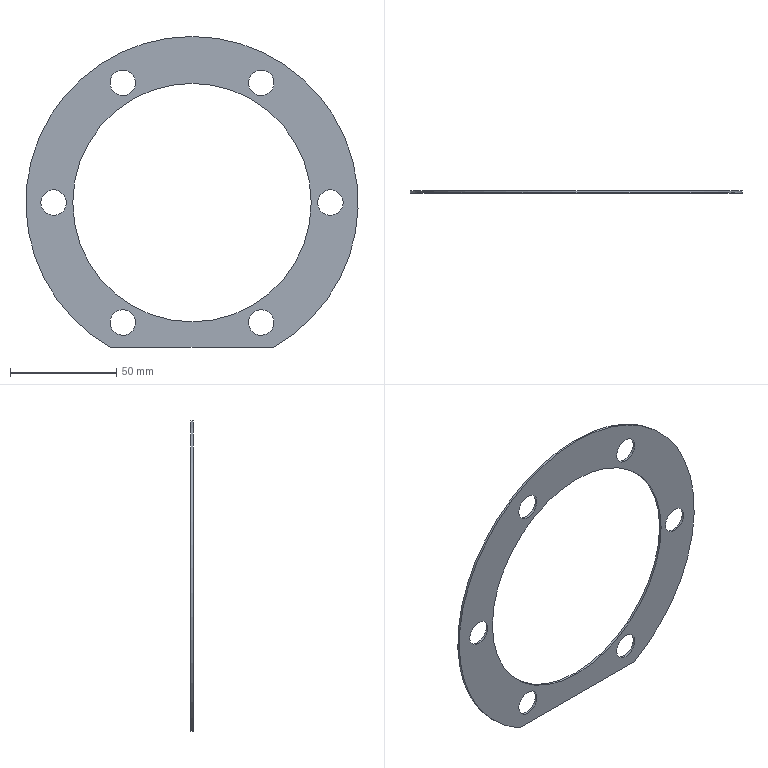Component | NX | T1_GASKET | 1 solid | 11 faces | box 156 x 1 x 146 mm | volume 8066 mm3 | cylinder 8 | plane 3 | commonest cylinder face diameters 12 x6 112 x1 156 x1
STEP:
#1=CARTESIAN_POINT('',(0.,0.,0.));
#2=DIRECTION('',(0.,0.,1.));
#3=DIRECTION('',(1.,0.,0.));
#4=AXIS2_PLACEMENT_3D('',#1,#2,#3);
#5=CARTESIAN_POINT('',(-41.21,121.,-71.));
#6=VERTEX_POINT('',#5);
#7=CARTESIAN_POINT('',(35.21,121.,-71.));
#8=VERTEX_POINT('',#7);
#9=CARTESIAN_POINT('',(-41.21,121.,-71.));
#10=DIRECTION('',(1.,0.,0.));
#11=VECTOR('',#10,1.);
#12=LINE('',#9,#11);
#13=CARTESIAN_POINT('',(-41.21,120.,-71.));
#14=DIRECTION('',(0.,0.,1.));
#15=DIRECTION('',(1.,0.,0.));
#16=AXIS2_PLACEMENT_3D('',#13,#14,#15);
#17=PLANE('',#16);
#18=CARTESIAN_POINT('',(0.,1.));
#19=DIRECTION('',(1.,0.));
#20=VECTOR('',#19,1.);
#21=LINE('',#18,#20);
#22=(GEOMETRIC_REPRESENTATION_CONTEXT(2)PARAMETRIC_REPRESENTATION_CONTEXT()REPRESENTATION_CONTEXT('',''));
#23=DEFINITIONAL_REPRESENTATION('',(#21),#22);
#24=PCURVE('',#17,#23);
#25=CARTESIAN_POINT('',(-3.,121.,-3.));
#26=DIRECTION('',(0.,-1.,0.));
#27=DIRECTION('',(0.,0.,-1.));
#28=AXIS2_PLACEMENT_3D('',#25,#26,#27);
#29=PLANE('',#28);
#30=CARTESIAN_POINT('',(68.,-38.21));
#31=DIRECTION('',(0.,1.));
#32=VECTOR('',#31,1.);
#33=LINE('',#30,#32);
#34=(GEOMETRIC_REPRESENTATION_CONTEXT(2)PARAMETRIC_REPRESENTATION_CONTEXT()REPRESENTATION_CONTEXT('',''));
#35=DEFINITIONAL_REPRESENTATION('',(#33),#34);
#36=PCURVE('',#29,#35);
#37=SURFACE_CURVE('',#12,(#24,#36),.PCURVE_S1.);
#38=EDGE_CURVE('',#6,#8,#37,.T.);
#39=ORIENTED_EDGE('',*,*,#38,.T.);
#40=CARTESIAN_POINT('',(35.21,120.,-71.));
#41=VERTEX_POINT('',#40);
#42=CARTESIAN_POINT('',(35.21,120.,-71.));
#43=DIRECTION('',(0.,1.,0.));
#44=VECTOR('',#43,1.);
#45=LINE('',#42,#44);
#46=CARTESIAN_POINT('',(76.42,0.));
#47=DIRECTION('',(0.,1.));
#48=VECTOR('',#47,1.);
#49=LINE('',#46,#48);
#50=(GEOMETRIC_REPRESENTATION_CONTEXT(2)PARAMETRIC_REPRESENTATION_CONTEXT()REPRESENTATION_CONTEXT('',''));
#51=DEFINITIONAL_REPRESENTATION('',(#49),#50);
#52=PCURVE('',#17,#51);
#53=CARTESIAN_POINT('',(-3.,120.,-3.));
#54=DIRECTION('',(0.,1.,0.));
#55=DIRECTION('',(0.,0.,1.));
#56=AXIS2_PLACEMENT_3D('',#53,#54,#55);
#57=CYLINDRICAL_SURFACE('',#56,78.);
#58=CARTESIAN_POINT('',(2.63,0.));
#59=DIRECTION('',(0.,1.));
#60=VECTOR('',#59,1.);
#61=LINE('',#58,#60);
#62=(GEOMETRIC_REPRESENTATION_CONTEXT(2)PARAMETRIC_REPRESENTATION_CONTEXT()REPRESENTATION_CONTEXT('',''));
#63=DEFINITIONAL_REPRESENTATION('',(#61),#62);
#64=PCURVE('',#57,#63);
#65=SURFACE_CURVE('',#45,(#52,#64),.PCURVE_S1.);
#66=EDGE_CURVE('',#41,#8,#65,.T.);
#67=ORIENTED_EDGE('',*,*,#66,.F.);
#68=CARTESIAN_POINT('',(-41.21,120.,-71.));
#69=VERTEX_POINT('',#68);
#70=CARTESIAN_POINT('',(-41.21,120.,-71.));
#71=DIRECTION('',(1.,0.,0.));
#72=VECTOR('',#71,1.);
#73=LINE('',#70,#72);
#74=CARTESIAN_POINT('',(0.,0.));
#75=DIRECTION('',(1.,0.));
#76=VECTOR('',#75,1.);
#77=LINE('',#74,#76);
#78=(GEOMETRIC_REPRESENTATION_CONTEXT(2)PARAMETRIC_REPRESENTATION_CONTEXT()REPRESENTATION_CONTEXT('',''));
#79=DEFINITIONAL_REPRESENTATION('',(#77),#78);
#80=PCURVE('',#17,#79);
#81=CARTESIAN_POINT('',(-3.,120.,-3.));
#82=DIRECTION('',(0.,-1.,0.));
#83=DIRECTION('',(0.,0.,-1.));
#84=AXIS2_PLACEMENT_3D('',#81,#82,#83);
#85=PLANE('',#84);
#86=CARTESIAN_POINT('',(68.,-38.21));
#87=DIRECTION('',(0.,1.));
#88=VECTOR('',#87,1.);
#89=LINE('',#86,#88);
#90=(GEOMETRIC_REPRESENTATION_CONTEXT(2)PARAMETRIC_REPRESENTATION_CONTEXT()REPRESENTATION_CONTEXT('',''));
#91=DEFINITIONAL_REPRESENTATION('',(#89),#90);
#92=PCURVE('',#85,#91);
#93=SURFACE_CURVE('',#73,(#80,#92),.PCURVE_S1.);
#94=EDGE_CURVE('',#69,#41,#93,.T.);
#95=ORIENTED_EDGE('',*,*,#94,.F.);
#96=CARTESIAN_POINT('',(-41.21,120.,-71.));
#97=DIRECTION('',(0.,-1.,0.));
#98=VECTOR('',#97,1.);
#99=LINE('',#96,#98);
#100=CARTESIAN_POINT('',(0.,0.));
#101=DIRECTION('',(0.,-1.));
#102=VECTOR('',#101,1.);
#103=LINE('',#100,#102);
#104=(GEOMETRIC_REPRESENTATION_CONTEXT(2)PARAMETRIC_REPRESENTATION_CONTEXT()REPRESENTATION_CONTEXT('',''));
#105=DEFINITIONAL_REPRESENTATION('',(#103),#104);
#106=PCURVE('',#17,#105);
#107=CARTESIAN_POINT('',(-2.63,0.));
#108=DIRECTION('',(0.,-1.));
#109=VECTOR('',#108,1.);
#110=LINE('',#107,#109);
#111=(GEOMETRIC_REPRESENTATION_CONTEXT(2)PARAMETRIC_REPRESENTATION_CONTEXT()REPRESENTATION_CONTEXT('',''));
#112=DEFINITIONAL_REPRESENTATION('',(#110),#111);
#113=PCURVE('',#57,#112);
#114=SURFACE_CURVE('',#99,(#106,#113),.PCURVE_S1.);
#115=EDGE_CURVE('',#6,#69,#114,.T.);
#116=ORIENTED_EDGE('',*,*,#115,.F.);
#117=EDGE_LOOP('',(#39,#67,#95,#116));
#118=FACE_BOUND('',#117,.T.);
#119=ADVANCED_FACE('',(#118),#17,.F.);
#120=CARTESIAN_POINT('',(32.5,120.,-64.488));
#121=VERTEX_POINT('',#120);
#122=CARTESIAN_POINT('',(29.5,120.,-59.292));
#123=DIRECTION('',(0.,-1.,0.));
#124=DIRECTION('',(0.5,0.,-0.866));
#125=AXIS2_PLACEMENT_3D('',#122,#123,#124);
#126=CIRCLE('',#125,6.);
#127=CARTESIAN_POINT('',(29.5,120.,-59.292));
#128=DIRECTION('',(0.,1.,0.));
#129=DIRECTION('',(0.,0.,1.));
#130=AXIS2_PLACEMENT_3D('',#127,#128,#129);
#131=CYLINDRICAL_SURFACE('',#130,6.);
#132=CARTESIAN_POINT('',(8.901,0.));
#133=DIRECTION('',(-1.,0.));
#134=VECTOR('',#133,1.);
#135=LINE('',#132,#134);
#136=(GEOMETRIC_REPRESENTATION_CONTEXT(2)PARAMETRIC_REPRESENTATION_CONTEXT()REPRESENTATION_CONTEXT('',''));
#137=DEFINITIONAL_REPRESENTATION('',(#135),#136);
#138=PCURVE('',#131,#137);
#139=CARTESIAN_POINT('',(56.292,32.5));
#140=DIRECTION('',(0.866,0.5));
#141=AXIS2_PLACEMENT_2D('',#139,#140);
#142=CIRCLE('',#141,6.);
#143=(GEOMETRIC_REPRESENTATION_CONTEXT(2)PARAMETRIC_REPRESENTATION_CONTEXT()REPRESENTATION_CONTEXT('',''));
#144=DEFINITIONAL_REPRESENTATION('',(#142),#143);
#145=PCURVE('',#85,#144);
#146=SURFACE_CURVE('',#126,(#138,#145),.PCURVE_S1.);
#147=EDGE_CURVE('',#121,#121,#146,.T.);
#148=ORIENTED_EDGE('',*,*,#147,.F.);
#149=CARTESIAN_POINT('',(32.5,121.,-64.488));
#150=VERTEX_POINT('',#149);
#151=CARTESIAN_POINT('',(32.5,120.,-64.488));
#152=CARTESIAN_POINT('',(32.5,121.,-64.488));
#153=B_SPLINE_CURVE_WITH_KNOTS('',1,(#151,#152),.UNSPECIFIED.,.F.,.F.,(2,2),(0.,1.),.PIECEWISE_BEZIER_KNOTS.);
#154=CARTESIAN_POINT('',(8.901,0.));
#155=DIRECTION('',(0.,1.));
#156=VECTOR('',#155,1.);
#157=LINE('',#154,#156);
#158=(GEOMETRIC_REPRESENTATION_CONTEXT(2)PARAMETRIC_REPRESENTATION_CONTEXT()REPRESENTATION_CONTEXT('',''));
#159=DEFINITIONAL_REPRESENTATION('',(#157),#158);
#160=PCURVE('',#131,#159);
#161=CARTESIAN_POINT('',(2.618,0.));
#162=DIRECTION('',(0.,1.));
#163=VECTOR('',#162,1.);
#164=LINE('',#161,#163);
#165=(GEOMETRIC_REPRESENTATION_CONTEXT(2)PARAMETRIC_REPRESENTATION_CONTEXT()REPRESENTATION_CONTEXT('',''));
#166=DEFINITIONAL_REPRESENTATION('',(#164),#165);
#167=PCURVE('',#131,#166);
#168=SEAM_CURVE('',#153,(#160,#167),.PCURVE_S1.);
#169=EDGE_CURVE('',#121,#150,#168,.T.);
#170=ORIENTED_EDGE('',*,*,#169,.T.);
#171=CARTESIAN_POINT('',(29.5,121.,-59.292));
#172=DIRECTION('',(0.,-1.,0.));
#173=DIRECTION('',(0.5,0.,-0.866));
#174=AXIS2_PLACEMENT_3D('',#171,#172,#173);
#175=CIRCLE('',#174,6.);
#176=CARTESIAN_POINT('',(8.901,1.));
#177=DIRECTION('',(-1.,0.));
#178=VECTOR('',#177,1.);
#179=LINE('',#176,#178);
#180=(GEOMETRIC_REPRESENTATION_CONTEXT(2)PARAMETRIC_REPRESENTATION_CONTEXT()REPRESENTATION_CONTEXT('',''));
#181=DEFINITIONAL_REPRESENTATION('',(#179),#180);
#182=PCURVE('',#131,#181);
#183=CARTESIAN_POINT('',(56.292,32.5));
#184=DIRECTION('',(0.866,0.5));
#185=AXIS2_PLACEMENT_2D('',#183,#184);
#186=CIRCLE('',#185,6.);
#187=(GEOMETRIC_REPRESENTATION_CONTEXT(2)PARAMETRIC_REPRESENTATION_CONTEXT()REPRESENTATION_CONTEXT('',''));
#188=DEFINITIONAL_REPRESENTATION('',(#186),#187);
#189=PCURVE('',#29,#188);
#190=SURFACE_CURVE('',#175,(#182,#189),.PCURVE_S1.);
#191=EDGE_CURVE('',#150,#150,#190,.T.);
#192=ORIENTED_EDGE('',*,*,#191,.T.);
#193=ORIENTED_EDGE('',*,*,#169,.F.);
#194=EDGE_LOOP('',(#148,#170,#192,#193));
#195=FACE_BOUND('',#194,.F.);
#196=ADVANCED_FACE('',(#195),#131,.F.);
#197=CARTESIAN_POINT('',(-38.5,120.,-64.488));
#198=VERTEX_POINT('',#197);
#199=CARTESIAN_POINT('',(-35.5,120.,-59.292));
#200=DIRECTION('',(0.,-1.,0.));
#201=DIRECTION('',(-0.5,0.,-0.866));
#202=AXIS2_PLACEMENT_3D('',#199,#200,#201);
#203=CIRCLE('',#202,6.);
#204=CARTESIAN_POINT('',(-35.5,120.,-59.292));
#205=DIRECTION('',(0.,1.,0.));
#206=DIRECTION('',(0.,0.,1.));
#207=AXIS2_PLACEMENT_3D('',#204,#205,#206);
#208=CYLINDRICAL_SURFACE('',#207,6.);
#209=CARTESIAN_POINT('',(9.948,0.));
#210=DIRECTION('',(-1.,0.));
#211=VECTOR('',#210,1.);
#212=LINE('',#209,#211);
#213=(GEOMETRIC_REPRESENTATION_CONTEXT(2)PARAMETRIC_REPRESENTATION_CONTEXT()REPRESENTATION_CONTEXT('',''));
#214=DEFINITIONAL_REPRESENTATION('',(#212),#213);
#215=PCURVE('',#208,#214);
#216=CARTESIAN_POINT('',(56.292,-32.5));
#217=DIRECTION('',(0.866,-0.5));
#218=AXIS2_PLACEMENT_2D('',#216,#217);
#219=CIRCLE('',#218,6.);
#220=(GEOMETRIC_REPRESENTATION_CONTEXT(2)PARAMETRIC_REPRESENTATION_CONTEXT()REPRESENTATION_CONTEXT('',''));
#221=DEFINITIONAL_REPRESENTATION('',(#219),#220);
#222=PCURVE('',#85,#221);
#223=SURFACE_CURVE('',#203,(#215,#222),.PCURVE_S1.);
#224=EDGE_CURVE('',#198,#198,#223,.T.);
#225=ORIENTED_EDGE('',*,*,#224,.F.);
#226=CARTESIAN_POINT('',(-38.5,121.,-64.488));
#227=VERTEX_POINT('',#226);
#228=CARTESIAN_POINT('',(-38.5,120.,-64.488));
#229=CARTESIAN_POINT('',(-38.5,121.,-64.488));
#230=B_SPLINE_CURVE_WITH_KNOTS('',1,(#228,#229),.UNSPECIFIED.,.F.,.F.,(2,2),(0.,1.),.PIECEWISE_BEZIER_KNOTS.);
#231=CARTESIAN_POINT('',(9.948,0.));
#232=DIRECTION('',(0.,1.));
#233=VECTOR('',#232,1.);
#234=LINE('',#231,#233);
#235=(GEOMETRIC_REPRESENTATION_CONTEXT(2)PARAMETRIC_REPRESENTATION_CONTEXT()REPRESENTATION_CONTEXT('',''));
#236=DEFINITIONAL_REPRESENTATION('',(#234),#235);
#237=PCURVE('',#208,#236);
#238=CARTESIAN_POINT('',(3.665,0.));
#239=DIRECTION('',(0.,1.));
#240=VECTOR('',#239,1.);
#241=LINE('',#238,#240);
#242=(GEOMETRIC_REPRESENTATION_CONTEXT(2)PARAMETRIC_REPRESENTATION_CONTEXT()REPRESENTATION_CONTEXT('',''));
#243=DEFINITIONAL_REPRESENTATION('',(#241),#242);
#244=PCURVE('',#208,#243);
#245=SEAM_CURVE('',#230,(#237,#244),.PCURVE_S1.);
#246=EDGE_CURVE('',#198,#227,#245,.T.);
#247=ORIENTED_EDGE('',*,*,#246,.T.);
#248=CARTESIAN_POINT('',(-35.5,121.,-59.292));
#249=DIRECTION('',(0.,-1.,0.));
#250=DIRECTION('',(-0.5,0.,-0.866));
#251=AXIS2_PLACEMENT_3D('',#248,#249,#250);
#252=CIRCLE('',#251,6.);
#253=CARTESIAN_POINT('',(9.948,1.));
#254=DIRECTION('',(-1.,0.));
#255=VECTOR('',#254,1.);
#256=LINE('',#253,#255);
#257=(GEOMETRIC_REPRESENTATION_CONTEXT(2)PARAMETRIC_REPRESENTATION_CONTEXT()REPRESENTATION_CONTEXT('',''));
#258=DEFINITIONAL_REPRESENTATION('',(#256),#257);
#259=PCURVE('',#208,#258);
#260=CARTESIAN_POINT('',(56.292,-32.5));
#261=DIRECTION('',(0.866,-0.5));
#262=AXIS2_PLACEMENT_2D('',#260,#261);
#263=CIRCLE('',#262,6.);
#264=(GEOMETRIC_REPRESENTATION_CONTEXT(2)PARAMETRIC_REPRESENTATION_CONTEXT()REPRESENTATION_CONTEXT('',''));
#265=DEFINITIONAL_REPRESENTATION('',(#263),#264);
#266=PCURVE('',#29,#265);
#267=SURFACE_CURVE('',#252,(#259,#266),.PCURVE_S1.);
#268=EDGE_CURVE('',#227,#227,#267,.T.);
#269=ORIENTED_EDGE('',*,*,#268,.T.);
#270=ORIENTED_EDGE('',*,*,#246,.F.);
#271=EDGE_LOOP('',(#225,#247,#269,#270));
#272=FACE_BOUND('',#271,.F.);
#273=ADVANCED_FACE('',(#272),#208,.F.);
#274=CARTESIAN_POINT('',(-74.,120.,-3.));
#275=VERTEX_POINT('',#274);
#276=CARTESIAN_POINT('',(-68.,120.,-3.));
#277=DIRECTION('',(0.,-1.,0.));
#278=DIRECTION('',(-1.,0.,0.));
#279=AXIS2_PLACEMENT_3D('',#276,#277,#278);
#280=CIRCLE('',#279,6.);
#281=CARTESIAN_POINT('',(-68.,120.,-3.));
#282=DIRECTION('',(0.,1.,0.));
#283=DIRECTION('',(0.,0.,1.));
#284=AXIS2_PLACEMENT_3D('',#281,#282,#283);
#285=CYLINDRICAL_SURFACE('',#284,6.);
#286=CARTESIAN_POINT('',(10.996,0.));
#287=DIRECTION('',(-1.,0.));
#288=VECTOR('',#287,1.);
#289=LINE('',#286,#288);
#290=(GEOMETRIC_REPRESENTATION_CONTEXT(2)PARAMETRIC_REPRESENTATION_CONTEXT()REPRESENTATION_CONTEXT('',''));
#291=DEFINITIONAL_REPRESENTATION('',(#289),#290);
#292=PCURVE('',#285,#291);
#293=CARTESIAN_POINT('',(0.,-65.));
#294=DIRECTION('',(-0.,-1.));
#295=AXIS2_PLACEMENT_2D('',#293,#294);
#296=CIRCLE('',#295,6.);
#297=(GEOMETRIC_REPRESENTATION_CONTEXT(2)PARAMETRIC_REPRESENTATION_CONTEXT()REPRESENTATION_CONTEXT('',''));
#298=DEFINITIONAL_REPRESENTATION('',(#296),#297);
#299=PCURVE('',#85,#298);
#300=SURFACE_CURVE('',#280,(#292,#299),.PCURVE_S1.);
#301=EDGE_CURVE('',#275,#275,#300,.T.);
#302=ORIENTED_EDGE('',*,*,#301,.F.);
#303=CARTESIAN_POINT('',(-74.,121.,-3.));
#304=VERTEX_POINT('',#303);
#305=CARTESIAN_POINT('',(-74.,120.,-3.));
#306=CARTESIAN_POINT('',(-74.,121.,-3.));
#307=B_SPLINE_CURVE_WITH_KNOTS('',1,(#305,#306),.UNSPECIFIED.,.F.,.F.,(2,2),(0.,1.),.PIECEWISE_BEZIER_KNOTS.);
#308=CARTESIAN_POINT('',(10.996,0.));
#309=DIRECTION('',(0.,1.));
#310=VECTOR('',#309,1.);
#311=LINE('',#308,#310);
#312=(GEOMETRIC_REPRESENTATION_CONTEXT(2)PARAMETRIC_REPRESENTATION_CONTEXT()REPRESENTATION_CONTEXT('',''));
#313=DEFINITIONAL_REPRESENTATION('',(#311),#312);
#314=PCURVE('',#285,#313);
#315=CARTESIAN_POINT('',(4.712,0.));
#316=DIRECTION('',(0.,1.));
#317=VECTOR('',#316,1.);
#318=LINE('',#315,#317);
#319=(GEOMETRIC_REPRESENTATION_CONTEXT(2)PARAMETRIC_REPRESENTATION_CONTEXT()REPRESENTATION_CONTEXT('',''));
#320=DEFINITIONAL_REPRESENTATION('',(#318),#319);
#321=PCURVE('',#285,#320);
#322=SEAM_CURVE('',#307,(#314,#321),.PCURVE_S1.);
#323=EDGE_CURVE('',#275,#304,#322,.T.);
#324=ORIENTED_EDGE('',*,*,#323,.T.);
#325=CARTESIAN_POINT('',(-68.,121.,-3.));
#326=DIRECTION('',(0.,-1.,0.));
#327=DIRECTION('',(-1.,0.,0.));
#328=AXIS2_PLACEMENT_3D('',#325,#326,#327);
#329=CIRCLE('',#328,6.);
#330=CARTESIAN_POINT('',(10.996,1.));
#331=DIRECTION('',(-1.,0.));
#332=VECTOR('',#331,1.);
#333=LINE('',#330,#332);
#334=(GEOMETRIC_REPRESENTATION_CONTEXT(2)PARAMETRIC_REPRESENTATION_CONTEXT()REPRESENTATION_CONTEXT('',''));
#335=DEFINITIONAL_REPRESENTATION('',(#333),#334);
#336=PCURVE('',#285,#335);
#337=CARTESIAN_POINT('',(0.,-65.));
#338=DIRECTION('',(-0.,-1.));
#339=AXIS2_PLACEMENT_2D('',#337,#338);
#340=CIRCLE('',#339,6.);
#341=(GEOMETRIC_REPRESENTATION_CONTEXT(2)PARAMETRIC_REPRESENTATION_CONTEXT()REPRESENTATION_CONTEXT('',''));
#342=DEFINITIONAL_REPRESENTATION('',(#340),#341);
#343=PCURVE('',#29,#342);
#344=SURFACE_CURVE('',#329,(#336,#343),.PCURVE_S1.);
#345=EDGE_CURVE('',#304,#304,#344,.T.);
#346=ORIENTED_EDGE('',*,*,#345,.T.);
#347=ORIENTED_EDGE('',*,*,#323,.F.);
#348=EDGE_LOOP('',(#302,#324,#346,#347));
#349=FACE_BOUND('',#348,.F.);
#350=ADVANCED_FACE('',(#349),#285,.F.);
#351=CARTESIAN_POINT('',(53.,120.,-3.));
#352=VERTEX_POINT('',#351);
#353=CARTESIAN_POINT('',(-3.,120.,-3.));
#354=DIRECTION('',(0.,-1.,0.));
#355=DIRECTION('',(1.,0.,-0.));
#356=AXIS2_PLACEMENT_3D('',#353,#354,#355);
#357=CIRCLE('',#356,56.);
#358=CARTESIAN_POINT('',(-3.,120.,-3.));
#359=DIRECTION('',(0.,1.,0.));
#360=DIRECTION('',(0.,0.,1.));
#361=AXIS2_PLACEMENT_3D('',#358,#359,#360);
#362=CYLINDRICAL_SURFACE('',#361,56.);
#363=CARTESIAN_POINT('',(7.854,0.));
#364=DIRECTION('',(-1.,0.));
#365=VECTOR('',#364,1.);
#366=LINE('',#363,#365);
#367=(GEOMETRIC_REPRESENTATION_CONTEXT(2)PARAMETRIC_REPRESENTATION_CONTEXT()REPRESENTATION_CONTEXT('',''));
#368=DEFINITIONAL_REPRESENTATION('',(#366),#367);
#369=PCURVE('',#362,#368);
#370=CARTESIAN_POINT('',(0.,0.));
#371=DIRECTION('',(0.,1.));
#372=AXIS2_PLACEMENT_2D('',#370,#371);
#373=CIRCLE('',#372,56.);
#374=(GEOMETRIC_REPRESENTATION_CONTEXT(2)PARAMETRIC_REPRESENTATION_CONTEXT()REPRESENTATION_CONTEXT('',''));
#375=DEFINITIONAL_REPRESENTATION('',(#373),#374);
#376=PCURVE('',#85,#375);
#377=SURFACE_CURVE('',#357,(#369,#376),.PCURVE_S1.);
#378=EDGE_CURVE('',#352,#352,#377,.T.);
#379=ORIENTED_EDGE('',*,*,#378,.F.);
#380=CARTESIAN_POINT('',(53.,121.,-3.));
#381=VERTEX_POINT('',#380);
#382=CARTESIAN_POINT('',(53.,120.,-3.));
#383=CARTESIAN_POINT('',(53.,121.,-3.));
#384=B_SPLINE_CURVE_WITH_KNOTS('',1,(#382,#383),.UNSPECIFIED.,.F.,.F.,(2,2),(0.,1.),.PIECEWISE_BEZIER_KNOTS.);
#385=CARTESIAN_POINT('',(7.854,0.));
#386=DIRECTION('',(0.,1.));
#387=VECTOR('',#386,1.);
#388=LINE('',#385,#387);
#389=(GEOMETRIC_REPRESENTATION_CONTEXT(2)PARAMETRIC_REPRESENTATION_CONTEXT()REPRESENTATION_CONTEXT('',''));
#390=DEFINITIONAL_REPRESENTATION('',(#388),#389);
#391=PCURVE('',#362,#390);
#392=CARTESIAN_POINT('',(1.571,0.));
#393=DIRECTION('',(0.,1.));
#394=VECTOR('',#393,1.);
#395=LINE('',#392,#394);
#396=(GEOMETRIC_REPRESENTATION_CONTEXT(2)PARAMETRIC_REPRESENTATION_CONTEXT()REPRESENTATION_CONTEXT('',''));
#397=DEFINITIONAL_REPRESENTATION('',(#395),#396);
#398=PCURVE('',#362,#397);
#399=SEAM_CURVE('',#384,(#391,#398),.PCURVE_S1.);
#400=EDGE_CURVE('',#352,#381,#399,.T.);
#401=ORIENTED_EDGE('',*,*,#400,.T.);
#402=CARTESIAN_POINT('',(-3.,121.,-3.));
#403=DIRECTION('',(0.,-1.,0.));
#404=DIRECTION('',(1.,0.,-0.));
#405=AXIS2_PLACEMENT_3D('',#402,#403,#404);
#406=CIRCLE('',#405,56.);
#407=CARTESIAN_POINT('',(7.854,1.));
#408=DIRECTION('',(-1.,0.));
#409=VECTOR('',#408,1.);
#410=LINE('',#407,#409);
#411=(GEOMETRIC_REPRESENTATION_CONTEXT(2)PARAMETRIC_REPRESENTATION_CONTEXT()REPRESENTATION_CONTEXT('',''));
#412=DEFINITIONAL_REPRESENTATION('',(#410),#411);
#413=PCURVE('',#362,#412);
#414=CARTESIAN_POINT('',(0.,0.));
#415=DIRECTION('',(0.,1.));
#416=AXIS2_PLACEMENT_2D('',#414,#415);
#417=CIRCLE('',#416,56.);
#418=(GEOMETRIC_REPRESENTATION_CONTEXT(2)PARAMETRIC_REPRESENTATION_CONTEXT()REPRESENTATION_CONTEXT('',''));
#419=DEFINITIONAL_REPRESENTATION('',(#417),#418);
#420=PCURVE('',#29,#419);
#421=SURFACE_CURVE('',#406,(#413,#420),.PCURVE_S1.);
#422=EDGE_CURVE('',#381,#381,#421,.T.);
#423=ORIENTED_EDGE('',*,*,#422,.T.);
#424=ORIENTED_EDGE('',*,*,#400,.F.);
#425=EDGE_LOOP('',(#379,#401,#423,#424));
#426=FACE_BOUND('',#425,.F.);
#427=ADVANCED_FACE('',(#426),#362,.F.);
#428=CARTESIAN_POINT('',(-38.5,120.,58.488));
#429=VERTEX_POINT('',#428);
#430=CARTESIAN_POINT('',(-35.5,120.,53.292));
#431=DIRECTION('',(0.,-1.,0.));
#432=DIRECTION('',(-0.5,0.,0.866));
#433=AXIS2_PLACEMENT_3D('',#430,#431,#432);
#434=CIRCLE('',#433,6.);
#435=CARTESIAN_POINT('',(-35.5,120.,53.292));
#436=DIRECTION('',(0.,1.,0.));
#437=DIRECTION('',(0.,0.,1.));
#438=AXIS2_PLACEMENT_3D('',#435,#436,#437);
#439=CYLINDRICAL_SURFACE('',#438,6.);
#440=CARTESIAN_POINT('',(12.043,0.));
#441=DIRECTION('',(-1.,0.));
#442=VECTOR('',#441,1.);
#443=LINE('',#440,#442);
#444=(GEOMETRIC_REPRESENTATION_CONTEXT(2)PARAMETRIC_REPRESENTATION_CONTEXT()REPRESENTATION_CONTEXT('',''));
#445=DEFINITIONAL_REPRESENTATION('',(#443),#444);
#446=PCURVE('',#439,#445);
#447=CARTESIAN_POINT('',(-56.292,-32.5));
#448=DIRECTION('',(-0.866,-0.5));
#449=AXIS2_PLACEMENT_2D('',#447,#448);
#450=CIRCLE('',#449,6.);
#451=(GEOMETRIC_REPRESENTATION_CONTEXT(2)PARAMETRIC_REPRESENTATION_CONTEXT()REPRESENTATION_CONTEXT('',''));
#452=DEFINITIONAL_REPRESENTATION('',(#450),#451);
#453=PCURVE('',#85,#452);
#454=SURFACE_CURVE('',#434,(#446,#453),.PCURVE_S1.);
#455=EDGE_CURVE('',#429,#429,#454,.T.);
#456=ORIENTED_EDGE('',*,*,#455,.F.);
#457=CARTESIAN_POINT('',(-38.5,121.,58.488));
#458=VERTEX_POINT('',#457);
#459=CARTESIAN_POINT('',(-38.5,120.,58.488));
#460=CARTESIAN_POINT('',(-38.5,121.,58.488));
#461=B_SPLINE_CURVE_WITH_KNOTS('',1,(#459,#460),.UNSPECIFIED.,.F.,.F.,(2,2),(0.,1.),.PIECEWISE_BEZIER_KNOTS.);
#462=CARTESIAN_POINT('',(12.043,0.));
#463=DIRECTION('',(0.,1.));
#464=VECTOR('',#463,1.);
#465=LINE('',#462,#464);
#466=(GEOMETRIC_REPRESENTATION_CONTEXT(2)PARAMETRIC_REPRESENTATION_CONTEXT()REPRESENTATION_CONTEXT('',''));
#467=DEFINITIONAL_REPRESENTATION('',(#465),#466);
#468=PCURVE('',#439,#467);
#469=CARTESIAN_POINT('',(5.76,0.));
#470=DIRECTION('',(0.,1.));
#471=VECTOR('',#470,1.);
#472=LINE('',#469,#471);
#473=(GEOMETRIC_REPRESENTATION_CONTEXT(2)PARAMETRIC_REPRESENTATION_CONTEXT()REPRESENTATION_CONTEXT('',''));
#474=DEFINITIONAL_REPRESENTATION('',(#472),#473);
#475=PCURVE('',#439,#474);
#476=SEAM_CURVE('',#461,(#468,#475),.PCURVE_S1.);
#477=EDGE_CURVE('',#429,#458,#476,.T.);
#478=ORIENTED_EDGE('',*,*,#477,.T.);
#479=CARTESIAN_POINT('',(-35.5,121.,53.292));
#480=DIRECTION('',(0.,-1.,0.));
#481=DIRECTION('',(-0.5,0.,0.866));
#482=AXIS2_PLACEMENT_3D('',#479,#480,#481);
#483=CIRCLE('',#482,6.);
#484=CARTESIAN_POINT('',(12.043,1.));
#485=DIRECTION('',(-1.,0.));
#486=VECTOR('',#485,1.);
#487=LINE('',#484,#486);
#488=(GEOMETRIC_REPRESENTATION_CONTEXT(2)PARAMETRIC_REPRESENTATION_CONTEXT()REPRESENTATION_CONTEXT('',''));
#489=DEFINITIONAL_REPRESENTATION('',(#487),#488);
#490=PCURVE('',#439,#489);
#491=CARTESIAN_POINT('',(-56.292,-32.5));
#492=DIRECTION('',(-0.866,-0.5));
#493=AXIS2_PLACEMENT_2D('',#491,#492);
#494=CIRCLE('',#493,6.);
#495=(GEOMETRIC_REPRESENTATION_CONTEXT(2)PARAMETRIC_REPRESENTATION_CONTEXT()REPRESENTATION_CONTEXT('',''));
#496=DEFINITIONAL_REPRESENTATION('',(#494),#495);
#497=PCURVE('',#29,#496);
#498=SURFACE_CURVE('',#483,(#490,#497),.PCURVE_S1.);
#499=EDGE_CURVE('',#458,#458,#498,.T.);
#500=ORIENTED_EDGE('',*,*,#499,.T.);
#501=ORIENTED_EDGE('',*,*,#477,.F.);
#502=EDGE_LOOP('',(#456,#478,#500,#501));
#503=FACE_BOUND('',#502,.F.);
#504=ADVANCED_FACE('',(#503),#439,.F.);
#505=CARTESIAN_POINT('',(32.5,120.,58.488));
#506=VERTEX_POINT('',#505);
#507=CARTESIAN_POINT('',(29.5,120.,53.292));
#508=DIRECTION('',(0.,-1.,0.));
#509=DIRECTION('',(0.5,0.,0.866));
#510=AXIS2_PLACEMENT_3D('',#507,#508,#509);
#511=CIRCLE('',#510,6.);
#512=CARTESIAN_POINT('',(29.5,120.,53.292));
#513=DIRECTION('',(0.,1.,0.));
#514=DIRECTION('',(0.,0.,1.));
#515=AXIS2_PLACEMENT_3D('',#512,#513,#514);
#516=CYLINDRICAL_SURFACE('',#515,6.);
#517=CARTESIAN_POINT('',(6.807,0.));
#518=DIRECTION('',(-1.,0.));
#519=VECTOR('',#518,1.);
#520=LINE('',#517,#519);
#521=(GEOMETRIC_REPRESENTATION_CONTEXT(2)PARAMETRIC_REPRESENTATION_CONTEXT()REPRESENTATION_CONTEXT('',''));
#522=DEFINITIONAL_REPRESENTATION('',(#520),#521);
#523=PCURVE('',#516,#522);
#524=CARTESIAN_POINT('',(-56.292,32.5));
#525=DIRECTION('',(-0.866,0.5));
#526=AXIS2_PLACEMENT_2D('',#524,#525);
#527=CIRCLE('',#526,6.);
#528=(GEOMETRIC_REPRESENTATION_CONTEXT(2)PARAMETRIC_REPRESENTATION_CONTEXT()REPRESENTATION_CONTEXT('',''));
#529=DEFINITIONAL_REPRESENTATION('',(#527),#528);
#530=PCURVE('',#85,#529);
#531=SURFACE_CURVE('',#511,(#523,#530),.PCURVE_S1.);
#532=EDGE_CURVE('',#506,#506,#531,.T.);
#533=ORIENTED_EDGE('',*,*,#532,.F.);
#534=CARTESIAN_POINT('',(32.5,121.,58.488));
#535=VERTEX_POINT('',#534);
#536=CARTESIAN_POINT('',(32.5,120.,58.488));
#537=CARTESIAN_POINT('',(32.5,121.,58.488));
#538=B_SPLINE_CURVE_WITH_KNOTS('',1,(#536,#537),.UNSPECIFIED.,.F.,.F.,(2,2),(0.,1.),.PIECEWISE_BEZIER_KNOTS.);
#539=CARTESIAN_POINT('',(6.807,0.));
#540=DIRECTION('',(0.,1.));
#541=VECTOR('',#540,1.);
#542=LINE('',#539,#541);
#543=(GEOMETRIC_REPRESENTATION_CONTEXT(2)PARAMETRIC_REPRESENTATION_CONTEXT()REPRESENTATION_CONTEXT('',''));
#544=DEFINITIONAL_REPRESENTATION('',(#542),#543);
#545=PCURVE('',#516,#544);
#546=CARTESIAN_POINT('',(0.5236,0.));
#547=DIRECTION('',(0.,1.));
#548=VECTOR('',#547,1.);
#549=LINE('',#546,#548);
#550=(GEOMETRIC_REPRESENTATION_CONTEXT(2)PARAMETRIC_REPRESENTATION_CONTEXT()REPRESENTATION_CONTEXT('',''));
#551=DEFINITIONAL_REPRESENTATION('',(#549),#550);
#552=PCURVE('',#516,#551);
#553=SEAM_CURVE('',#538,(#545,#552),.PCURVE_S1.);
#554=EDGE_CURVE('',#506,#535,#553,.T.);
#555=ORIENTED_EDGE('',*,*,#554,.T.);
#556=CARTESIAN_POINT('',(29.5,121.,53.292));
#557=DIRECTION('',(0.,-1.,0.));
#558=DIRECTION('',(0.5,0.,0.866));
#559=AXIS2_PLACEMENT_3D('',#556,#557,#558);
#560=CIRCLE('',#559,6.);
#561=CARTESIAN_POINT('',(6.807,1.));
#562=DIRECTION('',(-1.,0.));
#563=VECTOR('',#562,1.);
#564=LINE('',#561,#563);
#565=(GEOMETRIC_REPRESENTATION_CONTEXT(2)PARAMETRIC_REPRESENTATION_CONTEXT()REPRESENTATION_CONTEXT('',''));
#566=DEFINITIONAL_REPRESENTATION('',(#564),#565);
#567=PCURVE('',#516,#566);
#568=CARTESIAN_POINT('',(-56.292,32.5));
#569=DIRECTION('',(-0.866,0.5));
#570=AXIS2_PLACEMENT_2D('',#568,#569);
#571=CIRCLE('',#570,6.);
#572=(GEOMETRIC_REPRESENTATION_CONTEXT(2)PARAMETRIC_REPRESENTATION_CONTEXT()REPRESENTATION_CONTEXT('',''));
#573=DEFINITIONAL_REPRESENTATION('',(#571),#572);
#574=PCURVE('',#29,#573);
#575=SURFACE_CURVE('',#560,(#567,#574),.PCURVE_S1.);
#576=EDGE_CURVE('',#535,#535,#575,.T.);
#577=ORIENTED_EDGE('',*,*,#576,.T.);
#578=ORIENTED_EDGE('',*,*,#554,.F.);
#579=EDGE_LOOP('',(#533,#555,#577,#578));
#580=FACE_BOUND('',#579,.F.);
#581=ADVANCED_FACE('',(#580),#516,.F.);
#582=CARTESIAN_POINT('',(-3.,121.,-3.));
#583=DIRECTION('',(0.,-1.,0.));
#584=DIRECTION('',(1.,0.,-0.));
#585=AXIS2_PLACEMENT_3D('',#582,#583,#584);
#586=CIRCLE('',#585,78.);
#587=CARTESIAN_POINT('',(7.854,1.));
#588=DIRECTION('',(-1.,0.));
#589=VECTOR('',#588,1.);
#590=LINE('',#587,#589);
#591=(GEOMETRIC_REPRESENTATION_CONTEXT(2)PARAMETRIC_REPRESENTATION_CONTEXT()REPRESENTATION_CONTEXT('',''));
#592=DEFINITIONAL_REPRESENTATION('',(#590),#591);
#593=PCURVE('',#57,#592);
#594=CARTESIAN_POINT('',(0.,0.));
#595=DIRECTION('',(0.,1.));
#596=AXIS2_PLACEMENT_2D('',#594,#595);
#597=CIRCLE('',#596,78.);
#598=(GEOMETRIC_REPRESENTATION_CONTEXT(2)PARAMETRIC_REPRESENTATION_CONTEXT()REPRESENTATION_CONTEXT('',''));
#599=DEFINITIONAL_REPRESENTATION('',(#597),#598);
#600=PCURVE('',#29,#599);
#601=SURFACE_CURVE('',#586,(#593,#600),.PCURVE_S1.);
#602=EDGE_CURVE('',#8,#6,#601,.T.);
#603=ORIENTED_EDGE('',*,*,#602,.T.);
#604=ORIENTED_EDGE('',*,*,#115,.T.);
#605=CARTESIAN_POINT('',(-3.,120.,-3.));
#606=DIRECTION('',(0.,-1.,0.));
#607=DIRECTION('',(1.,0.,-0.));
#608=AXIS2_PLACEMENT_3D('',#605,#606,#607);
#609=CIRCLE('',#608,78.);
#610=CARTESIAN_POINT('',(7.854,0.));
#611=DIRECTION('',(-1.,0.));
#612=VECTOR('',#611,1.);
#613=LINE('',#610,#612);
#614=(GEOMETRIC_REPRESENTATION_CONTEXT(2)PARAMETRIC_REPRESENTATION_CONTEXT()REPRESENTATION_CONTEXT('',''));
#615=DEFINITIONAL_REPRESENTATION('',(#613),#614);
#616=PCURVE('',#57,#615);
#617=CARTESIAN_POINT('',(0.,0.));
#618=DIRECTION('',(0.,1.));
#619=AXIS2_PLACEMENT_2D('',#617,#618);
#620=CIRCLE('',#619,78.);
#621=(GEOMETRIC_REPRESENTATION_CONTEXT(2)PARAMETRIC_REPRESENTATION_CONTEXT()REPRESENTATION_CONTEXT('',''));
#622=DEFINITIONAL_REPRESENTATION('',(#620),#621);
#623=PCURVE('',#85,#622);
#624=SURFACE_CURVE('',#609,(#616,#623),.PCURVE_S1.);
#625=EDGE_CURVE('',#41,#69,#624,.T.);
#626=ORIENTED_EDGE('',*,*,#625,.F.);
#627=ORIENTED_EDGE('',*,*,#66,.T.);
#628=EDGE_LOOP('',(#603,#604,#626,#627));
#629=FACE_BOUND('',#628,.T.);
#630=ADVANCED_FACE('',(#629),#57,.T.);
#631=CARTESIAN_POINT('',(68.,120.,-3.));
#632=VERTEX_POINT('',#631);
#633=CARTESIAN_POINT('',(62.,120.,-3.));
#634=DIRECTION('',(0.,-1.,0.));
#635=DIRECTION('',(1.,0.,-0.));
#636=AXIS2_PLACEMENT_3D('',#633,#634,#635);
#637=CIRCLE('',#636,6.);
#638=CARTESIAN_POINT('',(62.,120.,-3.));
#639=DIRECTION('',(0.,1.,0.));
#640=DIRECTION('',(0.,0.,1.));
#641=AXIS2_PLACEMENT_3D('',#638,#639,#640);
#642=CYLINDRICAL_SURFACE('',#641,6.);
#643=CARTESIAN_POINT('',(7.854,0.));
#644=DIRECTION('',(-1.,0.));
#645=VECTOR('',#644,1.);
#646=LINE('',#643,#645);
#647=(GEOMETRIC_REPRESENTATION_CONTEXT(2)PARAMETRIC_REPRESENTATION_CONTEXT()REPRESENTATION_CONTEXT('',''));
#648=DEFINITIONAL_REPRESENTATION('',(#646),#647);
#649=PCURVE('',#642,#648);
#650=CARTESIAN_POINT('',(0.,65.));
#651=DIRECTION('',(0.,1.));
#652=AXIS2_PLACEMENT_2D('',#650,#651);
#653=CIRCLE('',#652,6.);
#654=(GEOMETRIC_REPRESENTATION_CONTEXT(2)PARAMETRIC_REPRESENTATION_CONTEXT()REPRESENTATION_CONTEXT('',''));
#655=DEFINITIONAL_REPRESENTATION('',(#653),#654);
#656=PCURVE('',#85,#655);
#657=SURFACE_CURVE('',#637,(#649,#656),.PCURVE_S1.);
#658=EDGE_CURVE('',#632,#632,#657,.T.);
#659=ORIENTED_EDGE('',*,*,#658,.F.);
#660=CARTESIAN_POINT('',(68.,121.,-3.));
#661=VERTEX_POINT('',#660);
#662=CARTESIAN_POINT('',(68.,120.,-3.));
#663=CARTESIAN_POINT('',(68.,121.,-3.));
#664=B_SPLINE_CURVE_WITH_KNOTS('',1,(#662,#663),.UNSPECIFIED.,.F.,.F.,(2,2),(0.,1.),.PIECEWISE_BEZIER_KNOTS.);
#665=CARTESIAN_POINT('',(7.854,0.));
#666=DIRECTION('',(0.,1.));
#667=VECTOR('',#666,1.);
#668=LINE('',#665,#667);
#669=(GEOMETRIC_REPRESENTATION_CONTEXT(2)PARAMETRIC_REPRESENTATION_CONTEXT()REPRESENTATION_CONTEXT('',''));
#670=DEFINITIONAL_REPRESENTATION('',(#668),#669);
#671=PCURVE('',#642,#670);
#672=CARTESIAN_POINT('',(1.571,0.));
#673=DIRECTION('',(0.,1.));
#674=VECTOR('',#673,1.);
#675=LINE('',#672,#674);
#676=(GEOMETRIC_REPRESENTATION_CONTEXT(2)PARAMETRIC_REPRESENTATION_CONTEXT()REPRESENTATION_CONTEXT('',''));
#677=DEFINITIONAL_REPRESENTATION('',(#675),#676);
#678=PCURVE('',#642,#677);
#679=SEAM_CURVE('',#664,(#671,#678),.PCURVE_S1.);
#680=EDGE_CURVE('',#632,#661,#679,.T.);
#681=ORIENTED_EDGE('',*,*,#680,.T.);
#682=CARTESIAN_POINT('',(62.,121.,-3.));
#683=DIRECTION('',(0.,-1.,0.));
#684=DIRECTION('',(1.,0.,-0.));
#685=AXIS2_PLACEMENT_3D('',#682,#683,#684);
#686=CIRCLE('',#685,6.);
#687=CARTESIAN_POINT('',(7.854,1.));
#688=DIRECTION('',(-1.,0.));
#689=VECTOR('',#688,1.);
#690=LINE('',#687,#689);
#691=(GEOMETRIC_REPRESENTATION_CONTEXT(2)PARAMETRIC_REPRESENTATION_CONTEXT()REPRESENTATION_CONTEXT('',''));
#692=DEFINITIONAL_REPRESENTATION('',(#690),#691);
#693=PCURVE('',#642,#692);
#694=CARTESIAN_POINT('',(0.,65.));
#695=DIRECTION('',(0.,1.));
#696=AXIS2_PLACEMENT_2D('',#694,#695);
#697=CIRCLE('',#696,6.);
#698=(GEOMETRIC_REPRESENTATION_CONTEXT(2)PARAMETRIC_REPRESENTATION_CONTEXT()REPRESENTATION_CONTEXT('',''));
#699=DEFINITIONAL_REPRESENTATION('',(#697),#698);
#700=PCURVE('',#29,#699);
#701=SURFACE_CURVE('',#686,(#693,#700),.PCURVE_S1.);
#702=EDGE_CURVE('',#661,#661,#701,.T.);
#703=ORIENTED_EDGE('',*,*,#702,.T.);
#704=ORIENTED_EDGE('',*,*,#680,.F.);
#705=EDGE_LOOP('',(#659,#681,#703,#704));
#706=FACE_BOUND('',#705,.F.);
#707=ADVANCED_FACE('',(#706),#642,.F.);
#708=ORIENTED_EDGE('',*,*,#94,.T.);
#709=ORIENTED_EDGE('',*,*,#625,.T.);
#710=EDGE_LOOP('',(#708,#709));
#711=FACE_BOUND('',#710,.T.);
#712=ORIENTED_EDGE('',*,*,#532,.F.);
#713=EDGE_LOOP('',(#712));
#714=FACE_BOUND('',#713,.T.);
#715=ORIENTED_EDGE('',*,*,#455,.F.);
#716=EDGE_LOOP('',(#715));
#717=FACE_BOUND('',#716,.T.);
#718=ORIENTED_EDGE('',*,*,#378,.F.);
#719=EDGE_LOOP('',(#718));
#720=FACE_BOUND('',#719,.T.);
#721=ORIENTED_EDGE('',*,*,#301,.F.);
#722=EDGE_LOOP('',(#721));
#723=FACE_BOUND('',#722,.T.);
#724=ORIENTED_EDGE('',*,*,#224,.F.);
#725=EDGE_LOOP('',(#724));
#726=FACE_BOUND('',#725,.T.);
#727=ORIENTED_EDGE('',*,*,#147,.F.);
#728=EDGE_LOOP('',(#727));
#729=FACE_BOUND('',#728,.T.);
#730=ORIENTED_EDGE('',*,*,#658,.F.);
#731=EDGE_LOOP('',(#730));
#732=FACE_BOUND('',#731,.T.);
#733=ADVANCED_FACE('',(#711,#714,#717,#720,#723,#726,#729,#732),#85,.T.);
#734=ORIENTED_EDGE('',*,*,#38,.F.);
#735=ORIENTED_EDGE('',*,*,#602,.F.);
#736=EDGE_LOOP('',(#734,#735));
#737=FACE_BOUND('',#736,.T.);
#738=ORIENTED_EDGE('',*,*,#576,.T.);
#739=EDGE_LOOP('',(#738));
#740=FACE_BOUND('',#739,.T.);
#741=ORIENTED_EDGE('',*,*,#499,.T.);
#742=EDGE_LOOP('',(#741));
#743=FACE_BOUND('',#742,.T.);
#744=ORIENTED_EDGE('',*,*,#422,.T.);
#745=EDGE_LOOP('',(#744));
#746=FACE_BOUND('',#745,.T.);
#747=ORIENTED_EDGE('',*,*,#345,.T.);
#748=EDGE_LOOP('',(#747));
#749=FACE_BOUND('',#748,.T.);
#750=ORIENTED_EDGE('',*,*,#268,.T.);
#751=EDGE_LOOP('',(#750));
#752=FACE_BOUND('',#751,.T.);
#753=ORIENTED_EDGE('',*,*,#191,.T.);
#754=EDGE_LOOP('',(#753));
#755=FACE_BOUND('',#754,.T.);
#756=ORIENTED_EDGE('',*,*,#702,.T.);
#757=EDGE_LOOP('',(#756));
#758=FACE_BOUND('',#757,.T.);
#759=ADVANCED_FACE('',(#737,#740,#743,#746,#749,#752,#755,#758),#29,.F.);
#760=CLOSED_SHELL('',(#119,#196,#273,#350,#427,#504,#581,#630,#707,#733,#759));
#761=MANIFOLD_SOLID_BREP('',#760);
#762=(LENGTH_UNIT()NAMED_UNIT(*)SI_UNIT(.MILLI.,.METRE.));
#763=UNCERTAINTY_MEASURE_WITH_UNIT(LENGTH_MEASURE(0.000005),#762,'','');
#764=(NAMED_UNIT(*)PLANE_ANGLE_UNIT()SI_UNIT($,.RADIAN.));
#765=(NAMED_UNIT(*)SI_UNIT($,.STERADIAN.)SOLID_ANGLE_UNIT());
#766=(GEOMETRIC_REPRESENTATION_CONTEXT(3)GLOBAL_UNCERTAINTY_ASSIGNED_CONTEXT((#763))GLOBAL_UNIT_ASSIGNED_CONTEXT((#762,#764,#765))REPRESENTATION_CONTEXT('',''));
#767=ADVANCED_BREP_SHAPE_REPRESENTATION('',(#4,#761),#766);